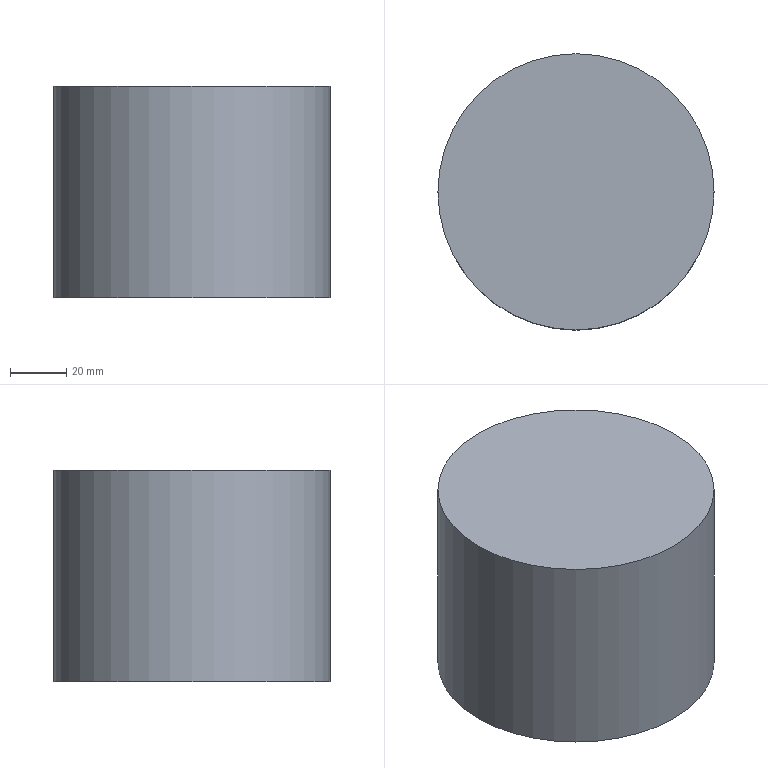Component | NX | TUBOGIRATORIO | 1 solid | 3 faces | box 98 x 98 x 75 mm | volume 565722 mm3 | plane 2 | cylinder 1 | commonest cylinder face diameters 98 x1
STEP:
#1=CARTESIAN_POINT('',(0.,0.,0.));
#2=DIRECTION('',(0.,0.,1.));
#3=DIRECTION('',(1.,0.,0.));
#4=AXIS2_PLACEMENT_3D('',#1,#2,#3);
#5=CARTESIAN_POINT('',(56.,-50.,-65.));
#6=VERTEX_POINT('',#5);
#7=CARTESIAN_POINT('',(154.,-50.,-65.));
#8=VERTEX_POINT('',#7);
#9=CARTESIAN_POINT('',(105.,-50.,-65.));
#10=DIRECTION('',(0.,0.,-1.));
#11=DIRECTION('',(-1.,0.,0.));
#12=AXIS2_PLACEMENT_3D('',#9,#10,#11);
#13=CIRCLE('',#12,49.);
#14=CARTESIAN_POINT('',(105.,-50.,-65.));
#15=DIRECTION('',(0.,0.,1.));
#16=DIRECTION('',(1.,0.,0.));
#17=AXIS2_PLACEMENT_3D('',#14,#15,#16);
#18=PLANE('',#17);
#19=CARTESIAN_POINT('',(-49.,0.));
#20=CARTESIAN_POINT('',(-49.,84.87));
#21=CARTESIAN_POINT('',(24.5,42.435));
#22=CARTESIAN_POINT('',(98.,0.));
#23=CARTESIAN_POINT('',(24.5,-42.435));
#24=CARTESIAN_POINT('',(-49.,-84.87));
#25=CARTESIAN_POINT('',(-49.,0.));
#26=(BOUNDED_CURVE()B_SPLINE_CURVE(2,(#19,#20,#21,#22,#23,#24,#25),.UNSPECIFIED.,.T.,.F.)B_SPLINE_CURVE_WITH_KNOTS((1,2,2,2,2,1),(-2.094,0.,2.094,4.189,6.283,8.378),.UNSPECIFIED.)CURVE()GEOMETRIC_REPRESENTATION_ITEM()RATIONAL_B_SPLINE_CURVE((1.,0.5,1.,0.5,1.,0.5,1.))REPRESENTATION_ITEM(''));
#27=(GEOMETRIC_REPRESENTATION_CONTEXT(2)PARAMETRIC_REPRESENTATION_CONTEXT()REPRESENTATION_CONTEXT('',''));
#28=DEFINITIONAL_REPRESENTATION('',(#26),#27);
#29=PCURVE('',#18,#28);
#30=CARTESIAN_POINT('',(105.,-50.,-140.));
#31=DIRECTION('',(0.,0.,1.));
#32=DIRECTION('',(1.,0.,0.));
#33=AXIS2_PLACEMENT_3D('',#30,#31,#32);
#34=CYLINDRICAL_SURFACE('',#33,49.);
#35=CARTESIAN_POINT('',(3.142,75.));
#36=DIRECTION('',(-1.,0.));
#37=VECTOR('',#36,1.);
#38=LINE('',#35,#37);
#39=(GEOMETRIC_REPRESENTATION_CONTEXT(2)PARAMETRIC_REPRESENTATION_CONTEXT()REPRESENTATION_CONTEXT('',''));
#40=DEFINITIONAL_REPRESENTATION('',(#38),#39);
#41=PCURVE('',#34,#40);
#42=SURFACE_CURVE('',#13,(#29,#41),.PCURVE_S1.);
#43=EDGE_CURVE('',#6,#8,#42,.T.);
#44=ORIENTED_EDGE('',*,*,#43,.F.);
#45=CARTESIAN_POINT('',(105.,-50.,-65.));
#46=DIRECTION('',(0.,0.,-1.));
#47=DIRECTION('',(-1.,0.,0.));
#48=AXIS2_PLACEMENT_3D('',#45,#46,#47);
#49=CIRCLE('',#48,49.);
#50=CARTESIAN_POINT('',(-49.,0.));
#51=CARTESIAN_POINT('',(-49.,84.87));
#52=CARTESIAN_POINT('',(24.5,42.435));
#53=CARTESIAN_POINT('',(98.,0.));
#54=CARTESIAN_POINT('',(24.5,-42.435));
#55=CARTESIAN_POINT('',(-49.,-84.87));
#56=CARTESIAN_POINT('',(-49.,0.));
#57=(BOUNDED_CURVE()B_SPLINE_CURVE(2,(#50,#51,#52,#53,#54,#55,#56),.UNSPECIFIED.,.T.,.F.)B_SPLINE_CURVE_WITH_KNOTS((1,2,2,2,2,1),(-2.094,0.,2.094,4.189,6.283,8.378),.UNSPECIFIED.)CURVE()GEOMETRIC_REPRESENTATION_ITEM()RATIONAL_B_SPLINE_CURVE((1.,0.5,1.,0.5,1.,0.5,1.))REPRESENTATION_ITEM(''));
#58=(GEOMETRIC_REPRESENTATION_CONTEXT(2)PARAMETRIC_REPRESENTATION_CONTEXT()REPRESENTATION_CONTEXT('',''));
#59=DEFINITIONAL_REPRESENTATION('',(#57),#58);
#60=PCURVE('',#18,#59);
#61=CARTESIAN_POINT('',(9.425,75.));
#62=DIRECTION('',(-1.,0.));
#63=VECTOR('',#62,1.);
#64=LINE('',#61,#63);
#65=(GEOMETRIC_REPRESENTATION_CONTEXT(2)PARAMETRIC_REPRESENTATION_CONTEXT()REPRESENTATION_CONTEXT('',''));
#66=DEFINITIONAL_REPRESENTATION('',(#64),#65);
#67=PCURVE('',#34,#66);
#68=SURFACE_CURVE('',#49,(#60,#67),.PCURVE_S1.);
#69=EDGE_CURVE('',#8,#6,#68,.T.);
#70=ORIENTED_EDGE('',*,*,#69,.F.);
#71=EDGE_LOOP('',(#44,#70));
#72=FACE_BOUND('',#71,.T.);
#73=ADVANCED_FACE('',(#72),#18,.T.);
#74=CARTESIAN_POINT('',(154.,-50.,-140.));
#75=VERTEX_POINT('',#74);
#76=CARTESIAN_POINT('',(105.,-50.,-140.));
#77=DIRECTION('',(0.,0.,1.));
#78=DIRECTION('',(1.,0.,0.));
#79=AXIS2_PLACEMENT_3D('',#76,#77,#78);
#80=CIRCLE('',#79,49.);
#81=CARTESIAN_POINT('',(105.,-50.,-140.));
#82=DIRECTION('',(0.,0.,-1.));
#83=DIRECTION('',(-1.,0.,0.));
#84=AXIS2_PLACEMENT_3D('',#81,#82,#83);
#85=PLANE('',#84);
#86=CARTESIAN_POINT('',(-49.,0.));
#87=CARTESIAN_POINT('',(-49.,84.87));
#88=CARTESIAN_POINT('',(24.5,42.435));
#89=CARTESIAN_POINT('',(98.,0.));
#90=CARTESIAN_POINT('',(24.5,-42.435));
#91=CARTESIAN_POINT('',(-49.,-84.87));
#92=CARTESIAN_POINT('',(-49.,0.));
#93=(BOUNDED_CURVE()B_SPLINE_CURVE(2,(#86,#87,#88,#89,#90,#91,#92),.UNSPECIFIED.,.T.,.F.)B_SPLINE_CURVE_WITH_KNOTS((1,2,2,2,2,1),(-2.094,0.,2.094,4.189,6.283,8.378),.UNSPECIFIED.)CURVE()GEOMETRIC_REPRESENTATION_ITEM()RATIONAL_B_SPLINE_CURVE((1.,0.5,1.,0.5,1.,0.5,1.))REPRESENTATION_ITEM(''));
#94=(GEOMETRIC_REPRESENTATION_CONTEXT(2)PARAMETRIC_REPRESENTATION_CONTEXT()REPRESENTATION_CONTEXT('',''));
#95=DEFINITIONAL_REPRESENTATION('',(#93),#94);
#96=PCURVE('',#85,#95);
#97=CARTESIAN_POINT('',(0.,0.));
#98=DIRECTION('',(1.,0.));
#99=VECTOR('',#98,1.);
#100=LINE('',#97,#99);
#101=(GEOMETRIC_REPRESENTATION_CONTEXT(2)PARAMETRIC_REPRESENTATION_CONTEXT()REPRESENTATION_CONTEXT('',''));
#102=DEFINITIONAL_REPRESENTATION('',(#100),#101);
#103=PCURVE('',#34,#102);
#104=SURFACE_CURVE('',#80,(#96,#103),.PCURVE_S1.);
#105=EDGE_CURVE('',#75,#75,#104,.T.);
#106=ORIENTED_EDGE('',*,*,#105,.F.);
#107=EDGE_LOOP('',(#106));
#108=FACE_BOUND('',#107,.T.);
#109=ADVANCED_FACE('',(#108),#85,.T.);
#110=ORIENTED_EDGE('',*,*,#43,.T.);
#111=CARTESIAN_POINT('',(154.,-50.,-140.));
#112=CARTESIAN_POINT('',(154.,-50.,-65.));
#113=B_SPLINE_CURVE_WITH_KNOTS('',1,(#111,#112),.UNSPECIFIED.,.F.,.F.,(2,2),(0.,75.),.PIECEWISE_BEZIER_KNOTS.);
#114=CARTESIAN_POINT('',(0.,0.));
#115=DIRECTION('',(0.,1.));
#116=VECTOR('',#115,1.);
#117=LINE('',#114,#116);
#118=(GEOMETRIC_REPRESENTATION_CONTEXT(2)PARAMETRIC_REPRESENTATION_CONTEXT()REPRESENTATION_CONTEXT('',''));
#119=DEFINITIONAL_REPRESENTATION('',(#117),#118);
#120=PCURVE('',#34,#119);
#121=CARTESIAN_POINT('',(6.283,0.));
#122=DIRECTION('',(0.,1.));
#123=VECTOR('',#122,1.);
#124=LINE('',#121,#123);
#125=(GEOMETRIC_REPRESENTATION_CONTEXT(2)PARAMETRIC_REPRESENTATION_CONTEXT()REPRESENTATION_CONTEXT('',''));
#126=DEFINITIONAL_REPRESENTATION('',(#124),#125);
#127=PCURVE('',#34,#126);
#128=SEAM_CURVE('',#113,(#120,#127),.PCURVE_S1.);
#129=EDGE_CURVE('',#75,#8,#128,.T.);
#130=ORIENTED_EDGE('',*,*,#129,.F.);
#131=ORIENTED_EDGE('',*,*,#105,.T.);
#132=ORIENTED_EDGE('',*,*,#129,.T.);
#133=ORIENTED_EDGE('',*,*,#69,.T.);
#134=EDGE_LOOP('',(#110,#130,#131,#132,#133));
#135=FACE_BOUND('',#134,.T.);
#136=ADVANCED_FACE('',(#135),#34,.T.);
#137=CLOSED_SHELL('',(#73,#109,#136));
#138=MANIFOLD_SOLID_BREP('',#137);
#139=(LENGTH_UNIT()NAMED_UNIT(*)SI_UNIT(.MILLI.,.METRE.));
#140=UNCERTAINTY_MEASURE_WITH_UNIT(LENGTH_MEASURE(0.000005),#139,'','');
#141=(NAMED_UNIT(*)PLANE_ANGLE_UNIT()SI_UNIT($,.RADIAN.));
#142=(NAMED_UNIT(*)SI_UNIT($,.STERADIAN.)SOLID_ANGLE_UNIT());
#143=(GEOMETRIC_REPRESENTATION_CONTEXT(3)GLOBAL_UNCERTAINTY_ASSIGNED_CONTEXT((#140))GLOBAL_UNIT_ASSIGNED_CONTEXT((#139,#141,#142))REPRESENTATION_CONTEXT('',''));
#144=ADVANCED_BREP_SHAPE_REPRESENTATION('',(#4,#138),#143);